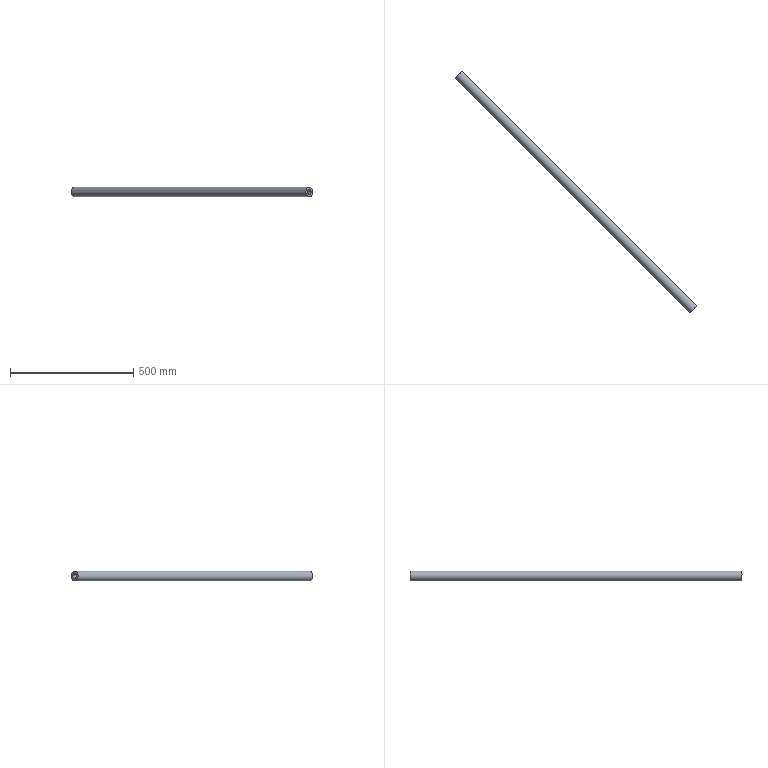Component | NX | SLIDING_POST | 1 solid | 4 faces | box 981.64 x 981.64 x 40 mm | volume 1270696 mm3 | plane 2 | cylinder 2 | commonest cylinder face diameters 40 x1 20 x1
STEP:
#1=CARTESIAN_POINT('',(0.,0.,0.));
#2=DIRECTION('',(0.,0.,1.));
#3=DIRECTION('',(1.,0.,0.));
#4=AXIS2_PLACEMENT_3D('',#1,#2,#3);
#5=CARTESIAN_POINT('',(-1280.009,1285.944,469.993));
#6=VERTEX_POINT('',#5);
#7=CARTESIAN_POINT('',(-1279.754,1286.199,460.));
#8=DIRECTION('',(-0.7071,0.7071,0.));
#9=DIRECTION('',(-0.02557,-0.02557,0.9993));
#10=AXIS2_PLACEMENT_3D('',#7,#8,#9);
#11=CIRCLE('',#10,10.);
#12=CARTESIAN_POINT('',(-1279.754,1286.199,460.));
#13=DIRECTION('',(-0.7071,0.7071,0.));
#14=DIRECTION('',(-0.02557,-0.02557,0.9993));
#15=AXIS2_PLACEMENT_3D('',#12,#13,#14);
#16=PLANE('',#15);
#17=CARTESIAN_POINT('',(0.,0.));
#18=DIRECTION('',(1.,-0.));
#19=AXIS2_PLACEMENT_2D('',#17,#18);
#20=CIRCLE('',#19,10.);
#21=(GEOMETRIC_REPRESENTATION_CONTEXT(2)PARAMETRIC_REPRESENTATION_CONTEXT()REPRESENTATION_CONTEXT('',''));
#22=DEFINITIONAL_REPRESENTATION('',(#20),#21);
#23=PCURVE('',#16,#22);
#24=CARTESIAN_POINT('',(-261.52,267.966,460.));
#25=DIRECTION('',(-0.7071,0.7071,0.));
#26=DIRECTION('',(-0.02557,-0.02557,0.9993));
#27=AXIS2_PLACEMENT_3D('',#24,#25,#26);
#28=CYLINDRICAL_SURFACE('',#27,10.);
#29=CARTESIAN_POINT('',(0.,1440.));
#30=DIRECTION('',(1.,0.));
#31=VECTOR('',#30,1.);
#32=LINE('',#29,#31);
#33=(GEOMETRIC_REPRESENTATION_CONTEXT(2)PARAMETRIC_REPRESENTATION_CONTEXT()REPRESENTATION_CONTEXT('',''));
#34=DEFINITIONAL_REPRESENTATION('',(#32),#33);
#35=PCURVE('',#28,#34);
#36=SURFACE_CURVE('',#11,(#23,#35),.PCURVE_S1.);
#37=EDGE_CURVE('',#6,#6,#36,.T.);
#38=ORIENTED_EDGE('',*,*,#37,.F.);
#39=EDGE_LOOP('',(#38));
#40=FACE_BOUND('',#39,.T.);
#41=CARTESIAN_POINT('',(-1280.265,1285.688,479.987));
#42=VERTEX_POINT('',#41);
#43=CARTESIAN_POINT('',(-1279.754,1286.199,460.));
#44=DIRECTION('',(0.7071,-0.7071,0.));
#45=DIRECTION('',(-0.02557,-0.02557,0.9993));
#46=AXIS2_PLACEMENT_3D('',#43,#44,#45);
#47=CIRCLE('',#46,20.);
#48=CARTESIAN_POINT('',(20.,0.));
#49=CARTESIAN_POINT('',(20.,-34.641));
#50=CARTESIAN_POINT('',(-10.,-17.321));
#51=CARTESIAN_POINT('',(-40.,-0.));
#52=CARTESIAN_POINT('',(-10.,17.321));
#53=CARTESIAN_POINT('',(20.,34.641));
#54=CARTESIAN_POINT('',(20.,0.));
#55=(BOUNDED_CURVE()B_SPLINE_CURVE(2,(#48,#49,#50,#51,#52,#53,#54),.UNSPECIFIED.,.T.,.F.)B_SPLINE_CURVE_WITH_KNOTS((1,2,2,2,2,1),(-2.094,0.,2.094,4.189,6.283,8.378),.UNSPECIFIED.)CURVE()GEOMETRIC_REPRESENTATION_ITEM()RATIONAL_B_SPLINE_CURVE((1.,0.5,1.,0.5,1.,0.5,1.))REPRESENTATION_ITEM(''));
#56=(GEOMETRIC_REPRESENTATION_CONTEXT(2)PARAMETRIC_REPRESENTATION_CONTEXT()REPRESENTATION_CONTEXT('',''));
#57=DEFINITIONAL_REPRESENTATION('',(#55),#56);
#58=PCURVE('',#16,#57);
#59=CARTESIAN_POINT('',(-326.397,332.843,460.));
#60=DIRECTION('',(-0.7071,0.7071,0.));
#61=DIRECTION('',(-0.02557,-0.02557,0.9993));
#62=AXIS2_PLACEMENT_3D('',#59,#60,#61);
#63=CYLINDRICAL_SURFACE('',#62,20.);
#64=CARTESIAN_POINT('',(6.283,1348.25));
#65=DIRECTION('',(-1.,0.));
#66=VECTOR('',#65,1.);
#67=LINE('',#64,#66);
#68=(GEOMETRIC_REPRESENTATION_CONTEXT(2)PARAMETRIC_REPRESENTATION_CONTEXT()REPRESENTATION_CONTEXT('',''));
#69=DEFINITIONAL_REPRESENTATION('',(#67),#68);
#70=PCURVE('',#63,#69);
#71=SURFACE_CURVE('',#47,(#58,#70),.PCURVE_S1.);
#72=EDGE_CURVE('',#42,#42,#71,.T.);
#73=ORIENTED_EDGE('',*,*,#72,.F.);
#74=EDGE_LOOP('',(#73));
#75=FACE_BOUND('',#74,.T.);
#76=ADVANCED_FACE('',(#40,#75),#16,.T.);
#77=CARTESIAN_POINT('',(-326.141,333.098,450.007));
#78=VERTEX_POINT('',#77);
#79=CARTESIAN_POINT('',(-326.653,332.587,469.993));
#80=VERTEX_POINT('',#79);
#81=CARTESIAN_POINT('',(-326.397,332.843,460.));
#82=DIRECTION('',(0.7071,-0.7071,0.));
#83=DIRECTION('',(0.02557,0.02557,-0.9993));
#84=AXIS2_PLACEMENT_3D('',#81,#82,#83);
#85=CIRCLE('',#84,10.);
#86=CARTESIAN_POINT('',(-326.397,332.843,460.));
#87=DIRECTION('',(0.7071,-0.7071,0.));
#88=DIRECTION('',(0.02557,0.02557,-0.9993));
#89=AXIS2_PLACEMENT_3D('',#86,#87,#88);
#90=PLANE('',#89);
#91=CARTESIAN_POINT('',(0.,0.));
#92=DIRECTION('',(1.,-0.));
#93=AXIS2_PLACEMENT_2D('',#91,#92);
#94=CIRCLE('',#93,10.);
#95=(GEOMETRIC_REPRESENTATION_CONTEXT(2)PARAMETRIC_REPRESENTATION_CONTEXT()REPRESENTATION_CONTEXT('',''));
#96=DEFINITIONAL_REPRESENTATION('',(#94),#95);
#97=PCURVE('',#90,#96);
#98=CARTESIAN_POINT('',(3.142,91.75));
#99=DIRECTION('',(-1.,0.));
#100=VECTOR('',#99,1.);
#101=LINE('',#98,#100);
#102=(GEOMETRIC_REPRESENTATION_CONTEXT(2)PARAMETRIC_REPRESENTATION_CONTEXT()REPRESENTATION_CONTEXT('',''));
#103=DEFINITIONAL_REPRESENTATION('',(#101),#102);
#104=PCURVE('',#28,#103);
#105=SURFACE_CURVE('',#85,(#97,#104),.PCURVE_S1.);
#106=EDGE_CURVE('',#78,#80,#105,.T.);
#107=ORIENTED_EDGE('',*,*,#106,.F.);
#108=CARTESIAN_POINT('',(-326.397,332.843,460.));
#109=DIRECTION('',(0.7071,-0.7071,0.));
#110=DIRECTION('',(0.02557,0.02557,-0.9993));
#111=AXIS2_PLACEMENT_3D('',#108,#109,#110);
#112=CIRCLE('',#111,10.);
#113=CARTESIAN_POINT('',(0.,0.));
#114=DIRECTION('',(1.,-0.));
#115=AXIS2_PLACEMENT_2D('',#113,#114);
#116=CIRCLE('',#115,10.);
#117=(GEOMETRIC_REPRESENTATION_CONTEXT(2)PARAMETRIC_REPRESENTATION_CONTEXT()REPRESENTATION_CONTEXT('',''));
#118=DEFINITIONAL_REPRESENTATION('',(#116),#117);
#119=PCURVE('',#90,#118);
#120=CARTESIAN_POINT('',(9.425,91.75));
#121=DIRECTION('',(-1.,0.));
#122=VECTOR('',#121,1.);
#123=LINE('',#120,#122);
#124=(GEOMETRIC_REPRESENTATION_CONTEXT(2)PARAMETRIC_REPRESENTATION_CONTEXT()REPRESENTATION_CONTEXT('',''));
#125=DEFINITIONAL_REPRESENTATION('',(#123),#124);
#126=PCURVE('',#28,#125);
#127=SURFACE_CURVE('',#112,(#119,#126),.PCURVE_S1.);
#128=EDGE_CURVE('',#80,#78,#127,.T.);
#129=ORIENTED_EDGE('',*,*,#128,.F.);
#130=EDGE_LOOP('',(#107,#129));
#131=FACE_BOUND('',#130,.T.);
#132=CARTESIAN_POINT('',(-326.908,332.331,479.987));
#133=VERTEX_POINT('',#132);
#134=CARTESIAN_POINT('',(-326.397,332.843,460.));
#135=DIRECTION('',(-0.7071,0.7071,0.));
#136=DIRECTION('',(-0.02557,-0.02557,0.9993));
#137=AXIS2_PLACEMENT_3D('',#134,#135,#136);
#138=CIRCLE('',#137,20.);
#139=CARTESIAN_POINT('',(-20.,0.));
#140=CARTESIAN_POINT('',(-20.,34.641));
#141=CARTESIAN_POINT('',(10.,17.321));
#142=CARTESIAN_POINT('',(40.,-0.));
#143=CARTESIAN_POINT('',(10.,-17.321));
#144=CARTESIAN_POINT('',(-20.,-34.641));
#145=CARTESIAN_POINT('',(-20.,0.));
#146=(BOUNDED_CURVE()B_SPLINE_CURVE(2,(#139,#140,#141,#142,#143,#144,#145),.UNSPECIFIED.,.T.,.F.)B_SPLINE_CURVE_WITH_KNOTS((1,2,2,2,2,1),(-2.094,0.,2.094,4.189,6.283,8.378),.UNSPECIFIED.)CURVE()GEOMETRIC_REPRESENTATION_ITEM()RATIONAL_B_SPLINE_CURVE((1.,0.5,1.,0.5,1.,0.5,1.))REPRESENTATION_ITEM(''));
#147=(GEOMETRIC_REPRESENTATION_CONTEXT(2)PARAMETRIC_REPRESENTATION_CONTEXT()REPRESENTATION_CONTEXT('',''));
#148=DEFINITIONAL_REPRESENTATION('',(#146),#147);
#149=PCURVE('',#90,#148);
#150=CARTESIAN_POINT('',(0.,0.));
#151=DIRECTION('',(1.,0.));
#152=VECTOR('',#151,1.);
#153=LINE('',#150,#152);
#154=(GEOMETRIC_REPRESENTATION_CONTEXT(2)PARAMETRIC_REPRESENTATION_CONTEXT()REPRESENTATION_CONTEXT('',''));
#155=DEFINITIONAL_REPRESENTATION('',(#153),#154);
#156=PCURVE('',#63,#155);
#157=SURFACE_CURVE('',#138,(#149,#156),.PCURVE_S1.);
#158=EDGE_CURVE('',#133,#133,#157,.T.);
#159=ORIENTED_EDGE('',*,*,#158,.F.);
#160=EDGE_LOOP('',(#159));
#161=FACE_BOUND('',#160,.T.);
#162=ADVANCED_FACE('',(#131,#161),#90,.T.);
#163=ORIENTED_EDGE('',*,*,#72,.T.);
#164=CARTESIAN_POINT('',(-326.908,332.331,479.987));
#165=CARTESIAN_POINT('',(-1280.265,1285.688,479.987));
#166=B_SPLINE_CURVE_WITH_KNOTS('',1,(#164,#165),.UNSPECIFIED.,.F.,.F.,(2,2),(0.,1348.25),.PIECEWISE_BEZIER_KNOTS.);
#167=CARTESIAN_POINT('',(0.,0.));
#168=DIRECTION('',(0.,1.));
#169=VECTOR('',#168,1.);
#170=LINE('',#167,#169);
#171=(GEOMETRIC_REPRESENTATION_CONTEXT(2)PARAMETRIC_REPRESENTATION_CONTEXT()REPRESENTATION_CONTEXT('',''));
#172=DEFINITIONAL_REPRESENTATION('',(#170),#171);
#173=PCURVE('',#63,#172);
#174=CARTESIAN_POINT('',(6.283,0.));
#175=DIRECTION('',(0.,1.));
#176=VECTOR('',#175,1.);
#177=LINE('',#174,#176);
#178=(GEOMETRIC_REPRESENTATION_CONTEXT(2)PARAMETRIC_REPRESENTATION_CONTEXT()REPRESENTATION_CONTEXT('',''));
#179=DEFINITIONAL_REPRESENTATION('',(#177),#178);
#180=PCURVE('',#63,#179);
#181=SEAM_CURVE('',#166,(#173,#180),.PCURVE_S1.);
#182=EDGE_CURVE('',#133,#42,#181,.T.);
#183=ORIENTED_EDGE('',*,*,#182,.F.);
#184=ORIENTED_EDGE('',*,*,#158,.T.);
#185=ORIENTED_EDGE('',*,*,#182,.T.);
#186=EDGE_LOOP('',(#163,#183,#184,#185));
#187=FACE_BOUND('',#186,.T.);
#188=ADVANCED_FACE('',(#187),#63,.T.);
#189=ORIENTED_EDGE('',*,*,#128,.F.);
#190=CARTESIAN_POINT('',(-326.653,332.587,469.993));
#191=CARTESIAN_POINT('',(-1280.009,1285.944,469.993));
#192=B_SPLINE_CURVE_WITH_KNOTS('',1,(#190,#191),.UNSPECIFIED.,.F.,.F.,(2,2),(91.75,1440.),.PIECEWISE_BEZIER_KNOTS.);
#193=CARTESIAN_POINT('',(6.283,0.));
#194=DIRECTION('',(0.,1.));
#195=VECTOR('',#194,1.);
#196=LINE('',#193,#195);
#197=(GEOMETRIC_REPRESENTATION_CONTEXT(2)PARAMETRIC_REPRESENTATION_CONTEXT()REPRESENTATION_CONTEXT('',''));
#198=DEFINITIONAL_REPRESENTATION('',(#196),#197);
#199=PCURVE('',#28,#198);
#200=CARTESIAN_POINT('',(0.,0.));
#201=DIRECTION('',(0.,1.));
#202=VECTOR('',#201,1.);
#203=LINE('',#200,#202);
#204=(GEOMETRIC_REPRESENTATION_CONTEXT(2)PARAMETRIC_REPRESENTATION_CONTEXT()REPRESENTATION_CONTEXT('',''));
#205=DEFINITIONAL_REPRESENTATION('',(#203),#204);
#206=PCURVE('',#28,#205);
#207=SEAM_CURVE('',#192,(#199,#206),.PCURVE_S1.);
#208=EDGE_CURVE('',#80,#6,#207,.T.);
#209=ORIENTED_EDGE('',*,*,#208,.T.);
#210=ORIENTED_EDGE('',*,*,#37,.F.);
#211=ORIENTED_EDGE('',*,*,#208,.F.);
#212=ORIENTED_EDGE('',*,*,#106,.F.);
#213=EDGE_LOOP('',(#189,#209,#210,#211,#212));
#214=FACE_BOUND('',#213,.F.);
#215=ADVANCED_FACE('',(#214),#28,.F.);
#216=CLOSED_SHELL('',(#76,#162,#188,#215));
#217=MANIFOLD_SOLID_BREP('',#216);
#218=(LENGTH_UNIT()NAMED_UNIT(*)SI_UNIT(.MILLI.,.METRE.));
#219=UNCERTAINTY_MEASURE_WITH_UNIT(LENGTH_MEASURE(0.000005),#218,'','');
#220=(NAMED_UNIT(*)PLANE_ANGLE_UNIT()SI_UNIT($,.RADIAN.));
#221=(NAMED_UNIT(*)SI_UNIT($,.STERADIAN.)SOLID_ANGLE_UNIT());
#222=(GEOMETRIC_REPRESENTATION_CONTEXT(3)GLOBAL_UNCERTAINTY_ASSIGNED_CONTEXT((#219))GLOBAL_UNIT_ASSIGNED_CONTEXT((#218,#220,#221))REPRESENTATION_CONTEXT('',''));
#223=ADVANCED_BREP_SHAPE_REPRESENTATION('',(#4,#217),#222);